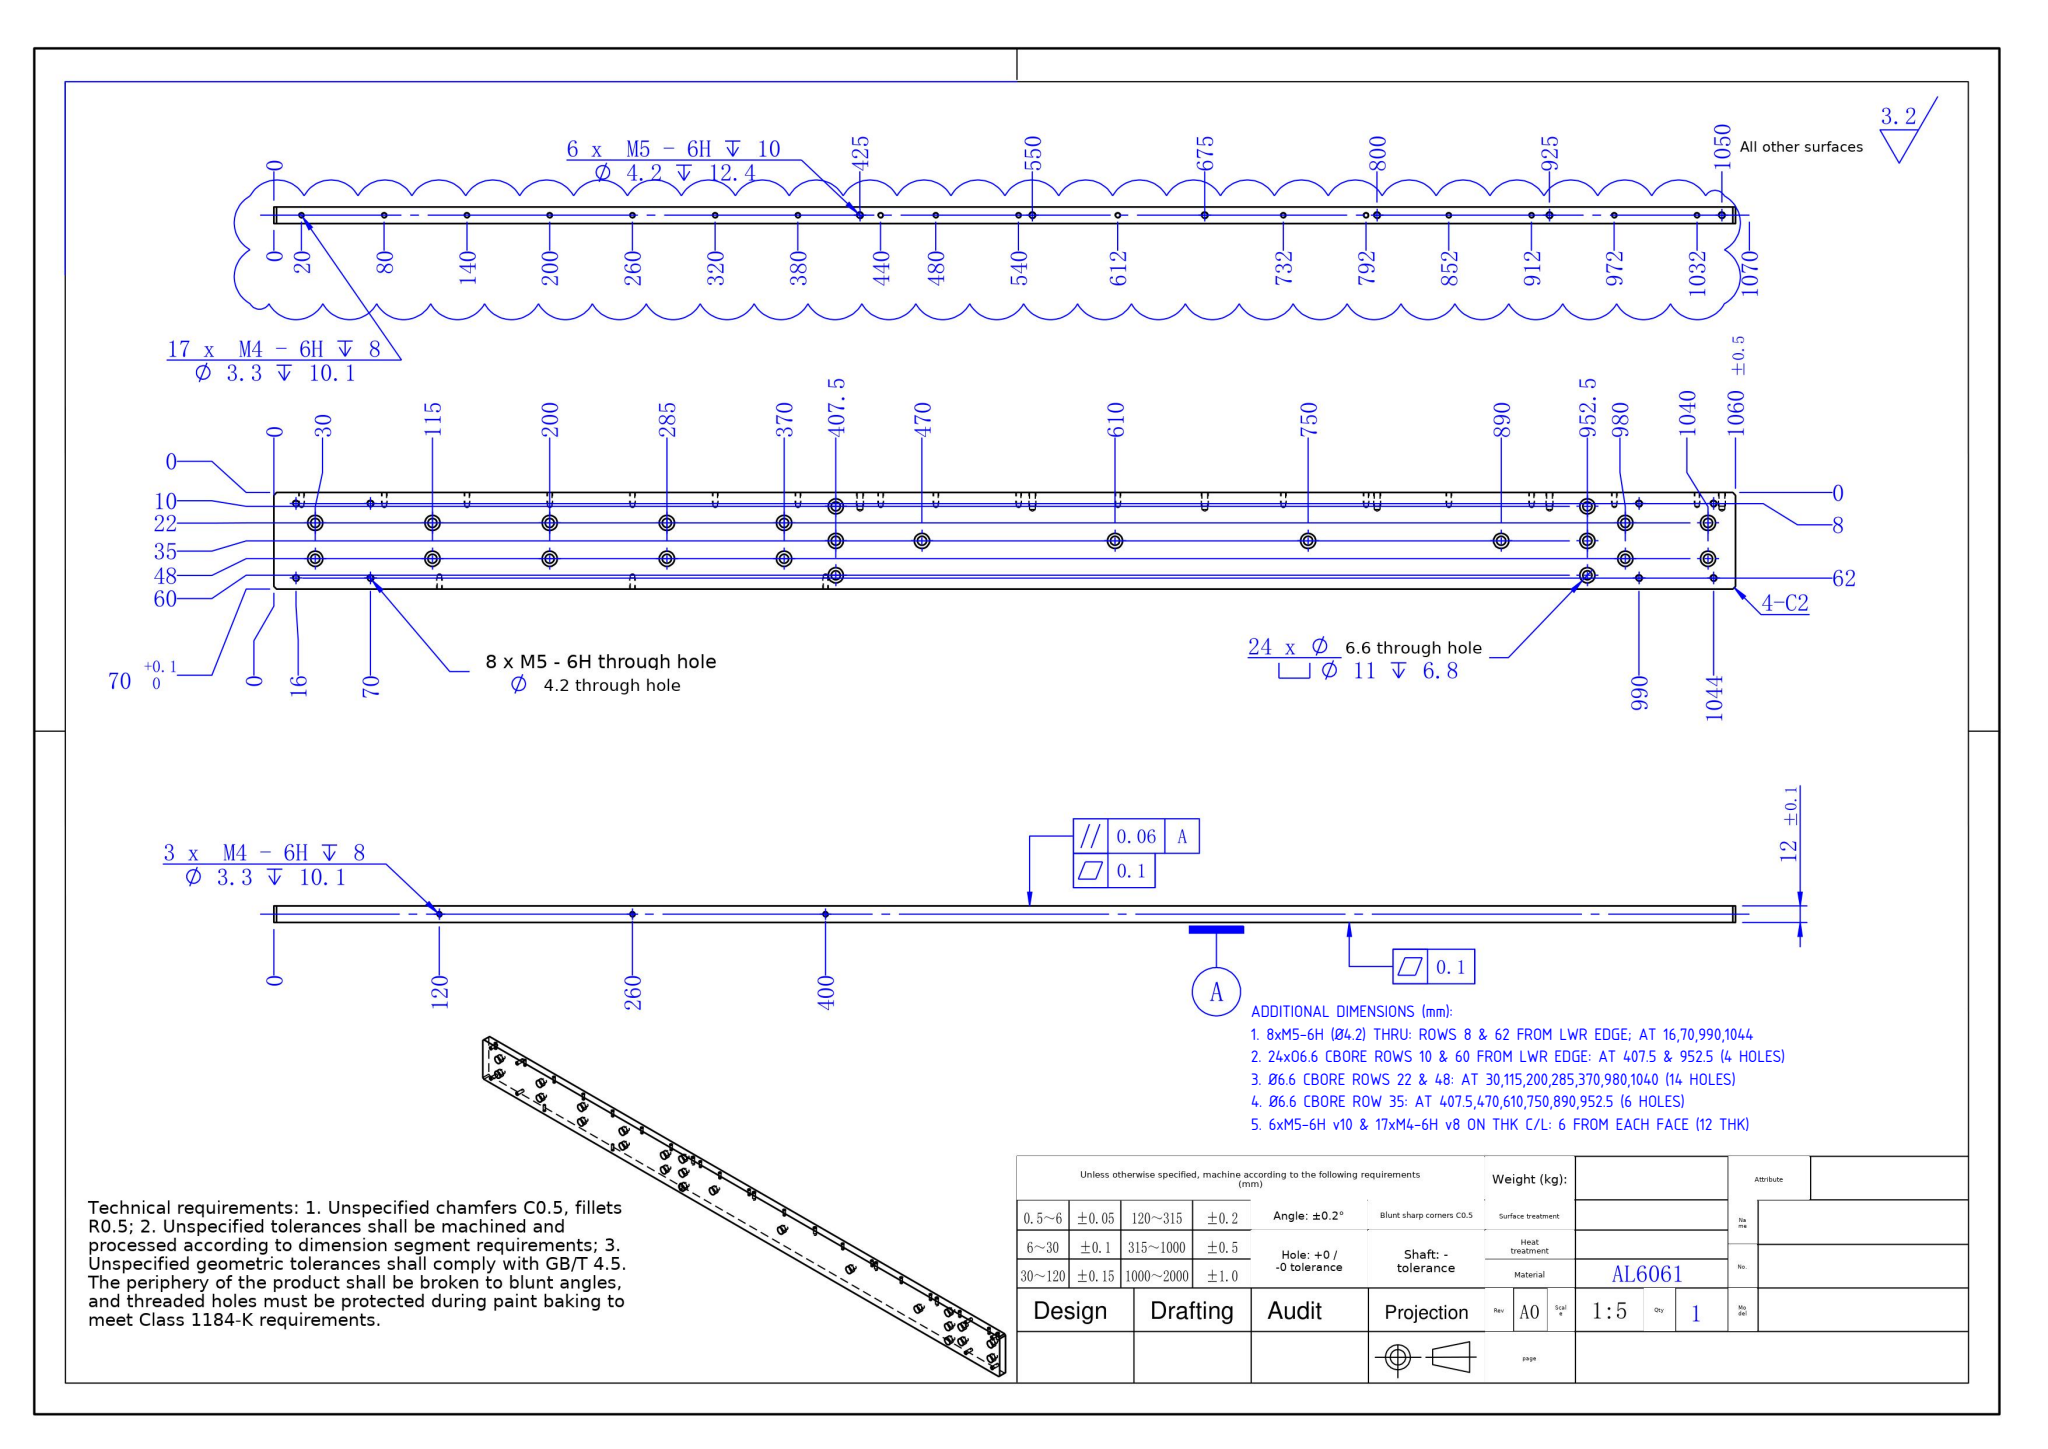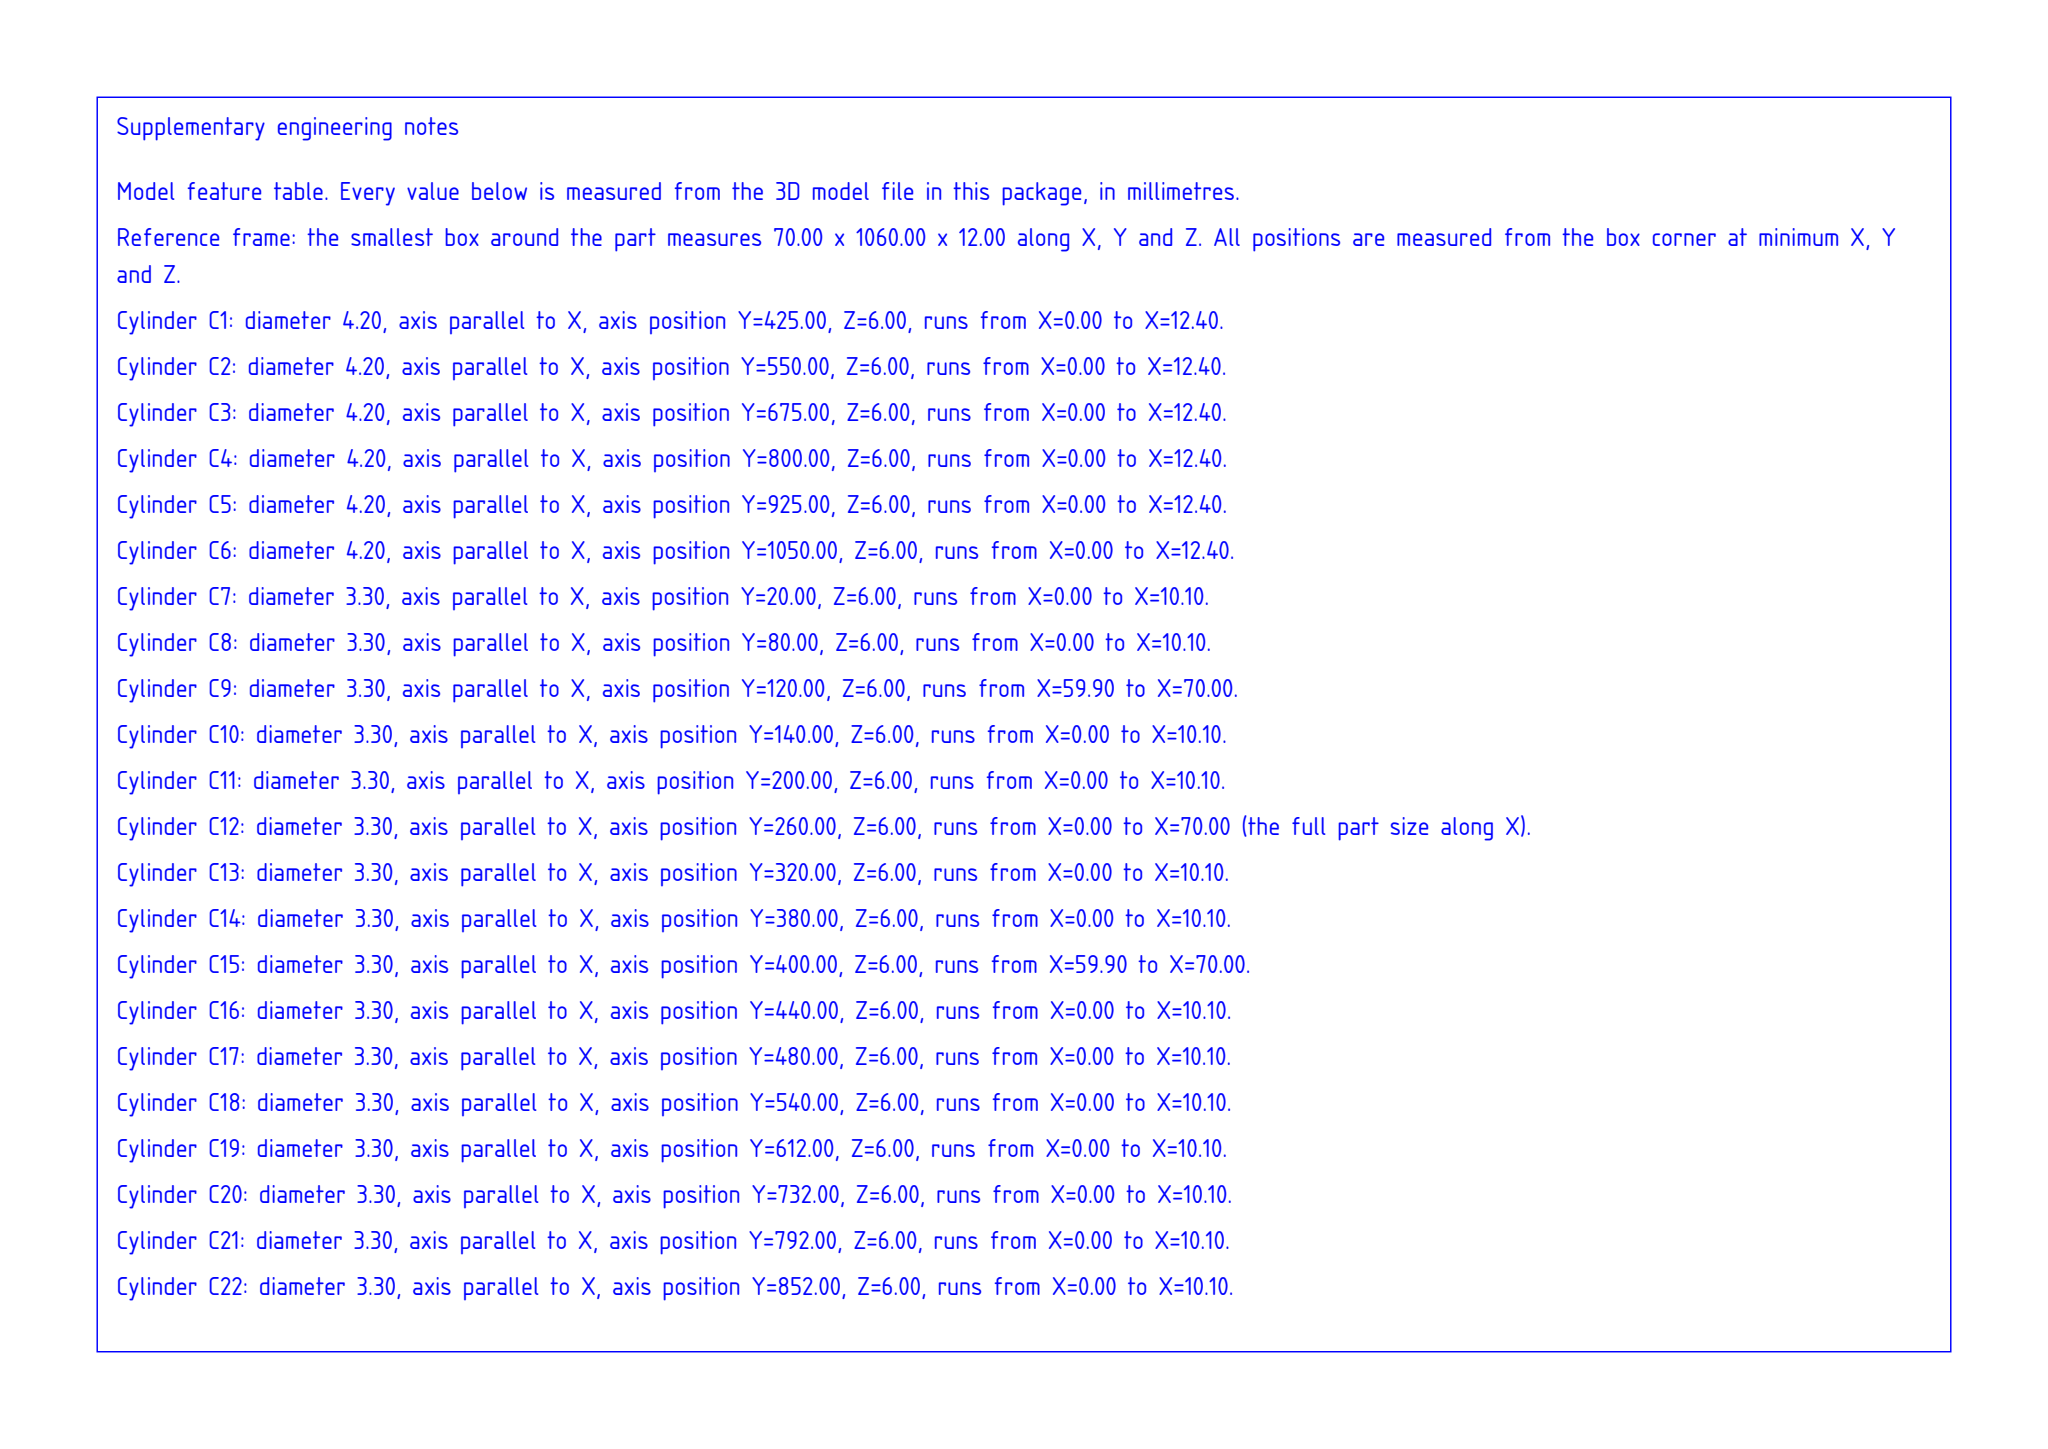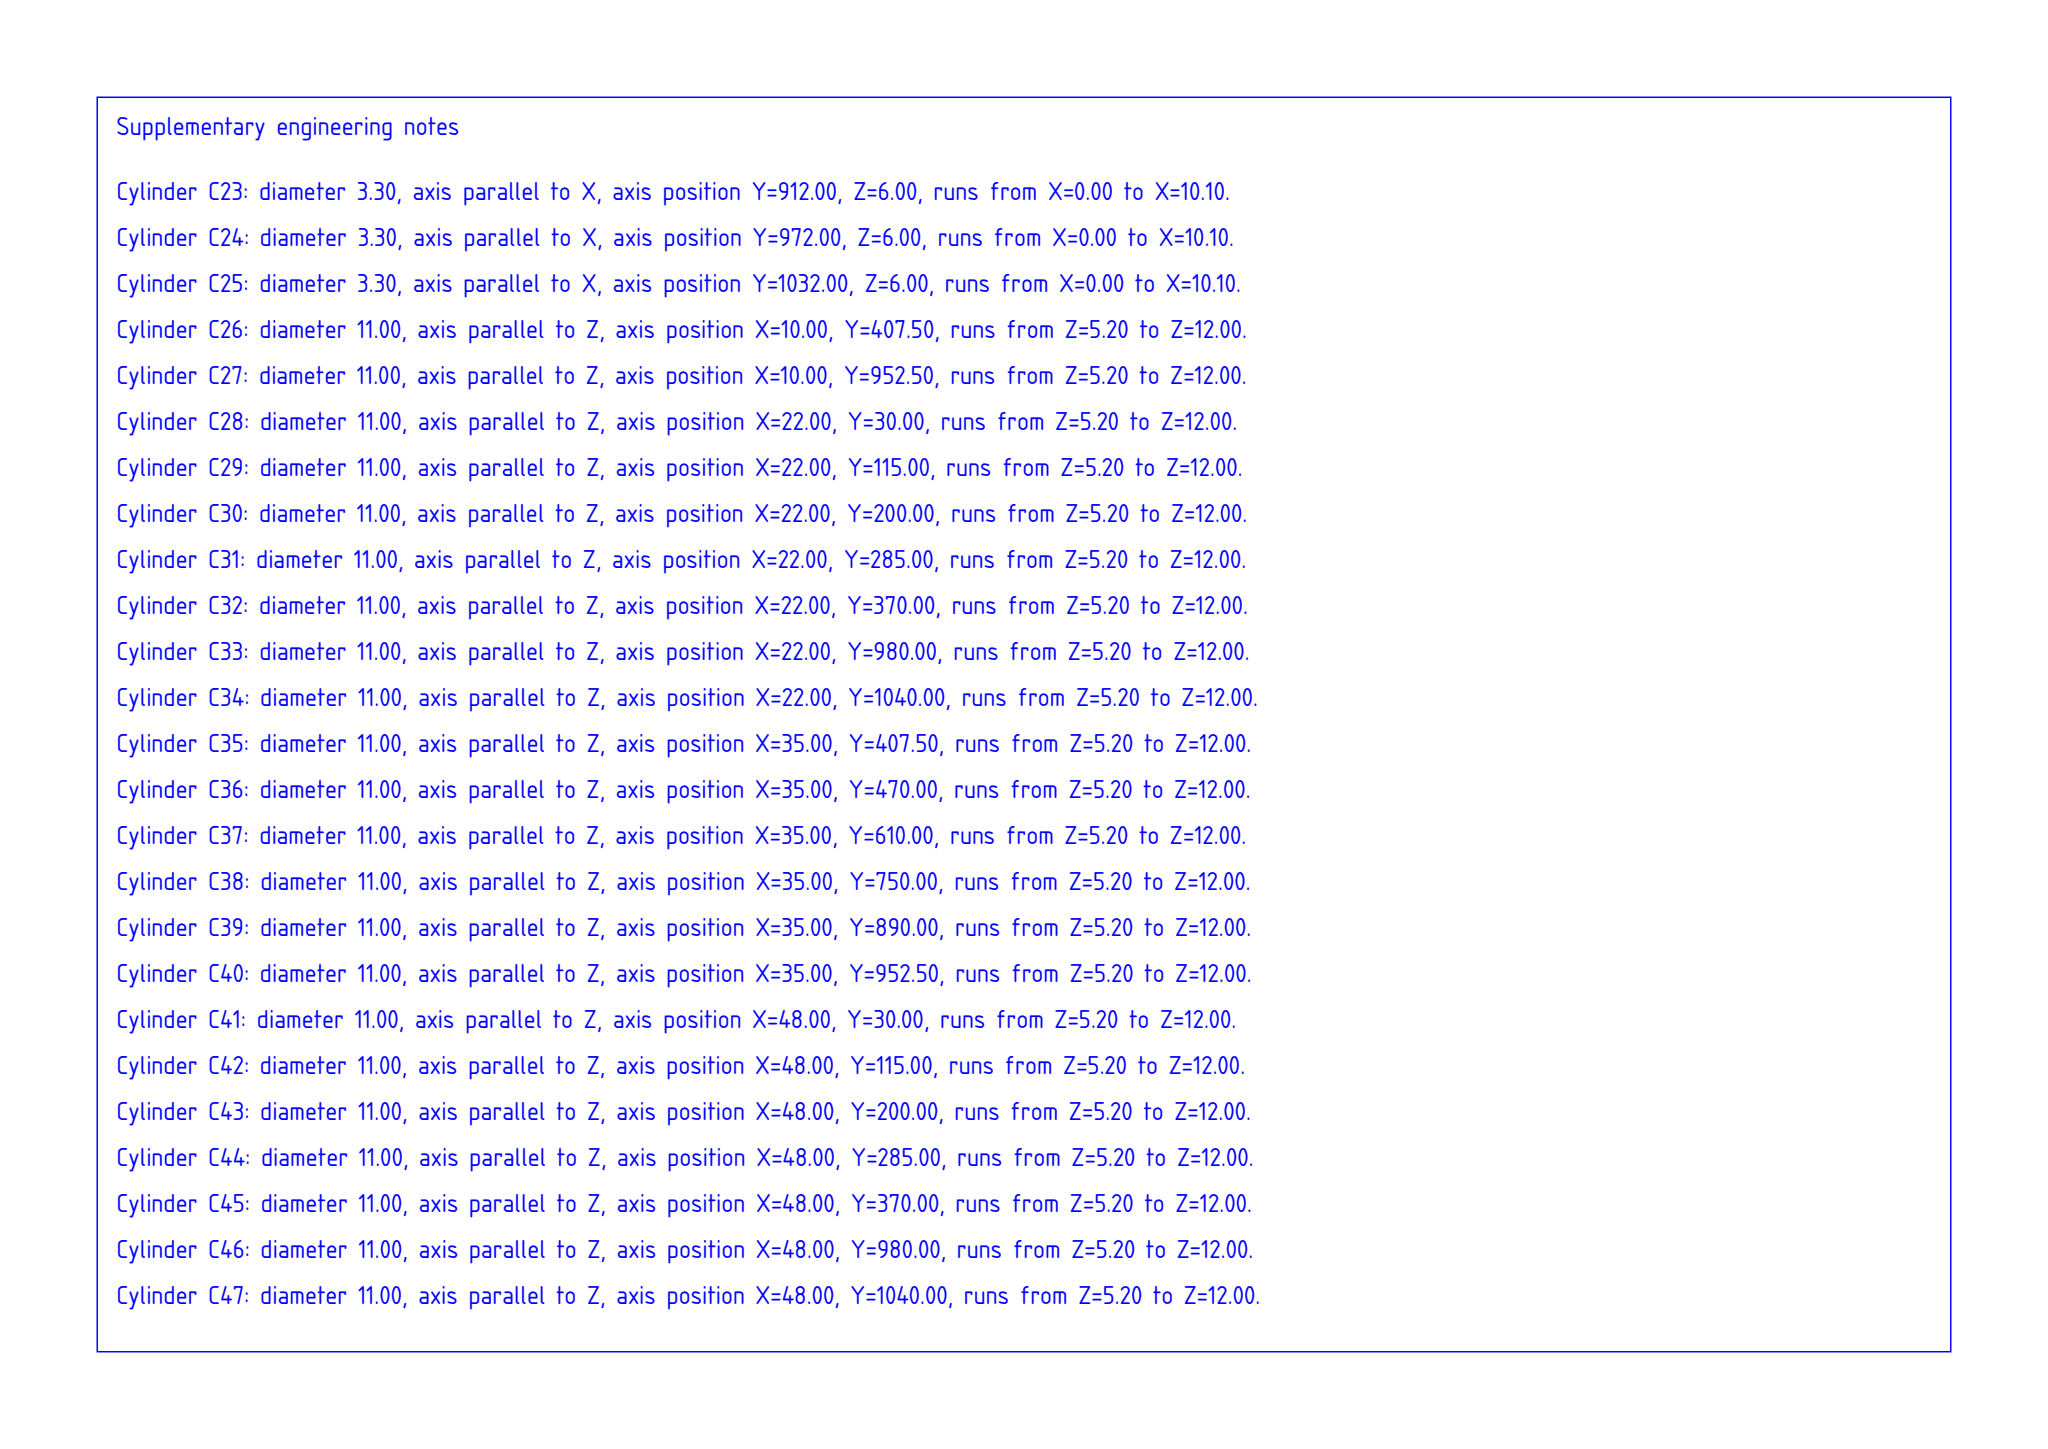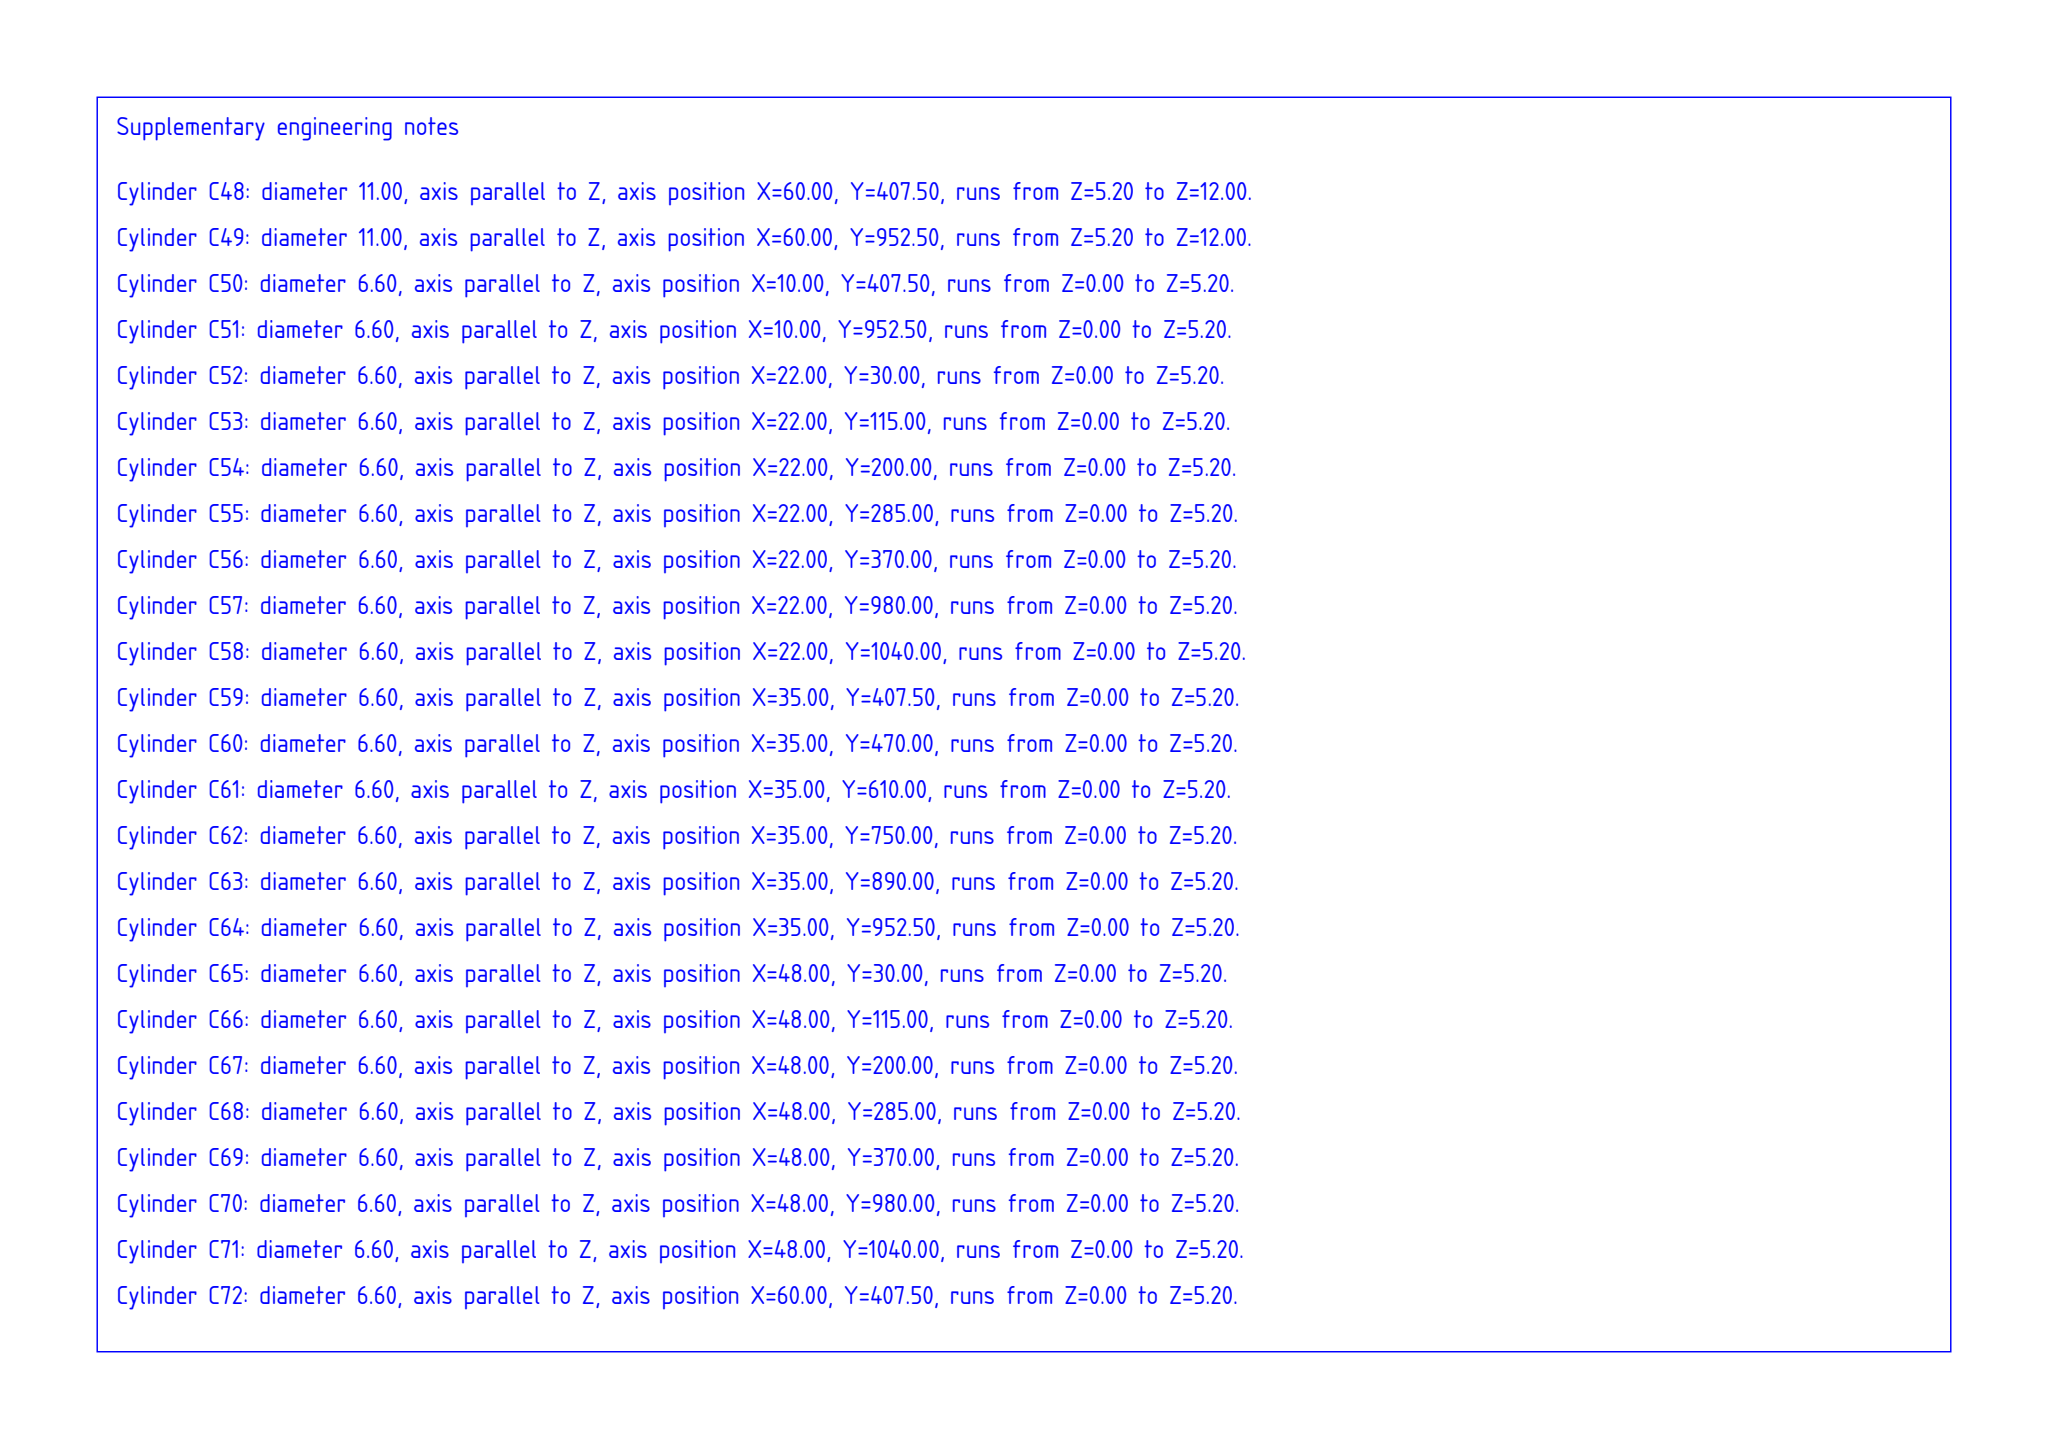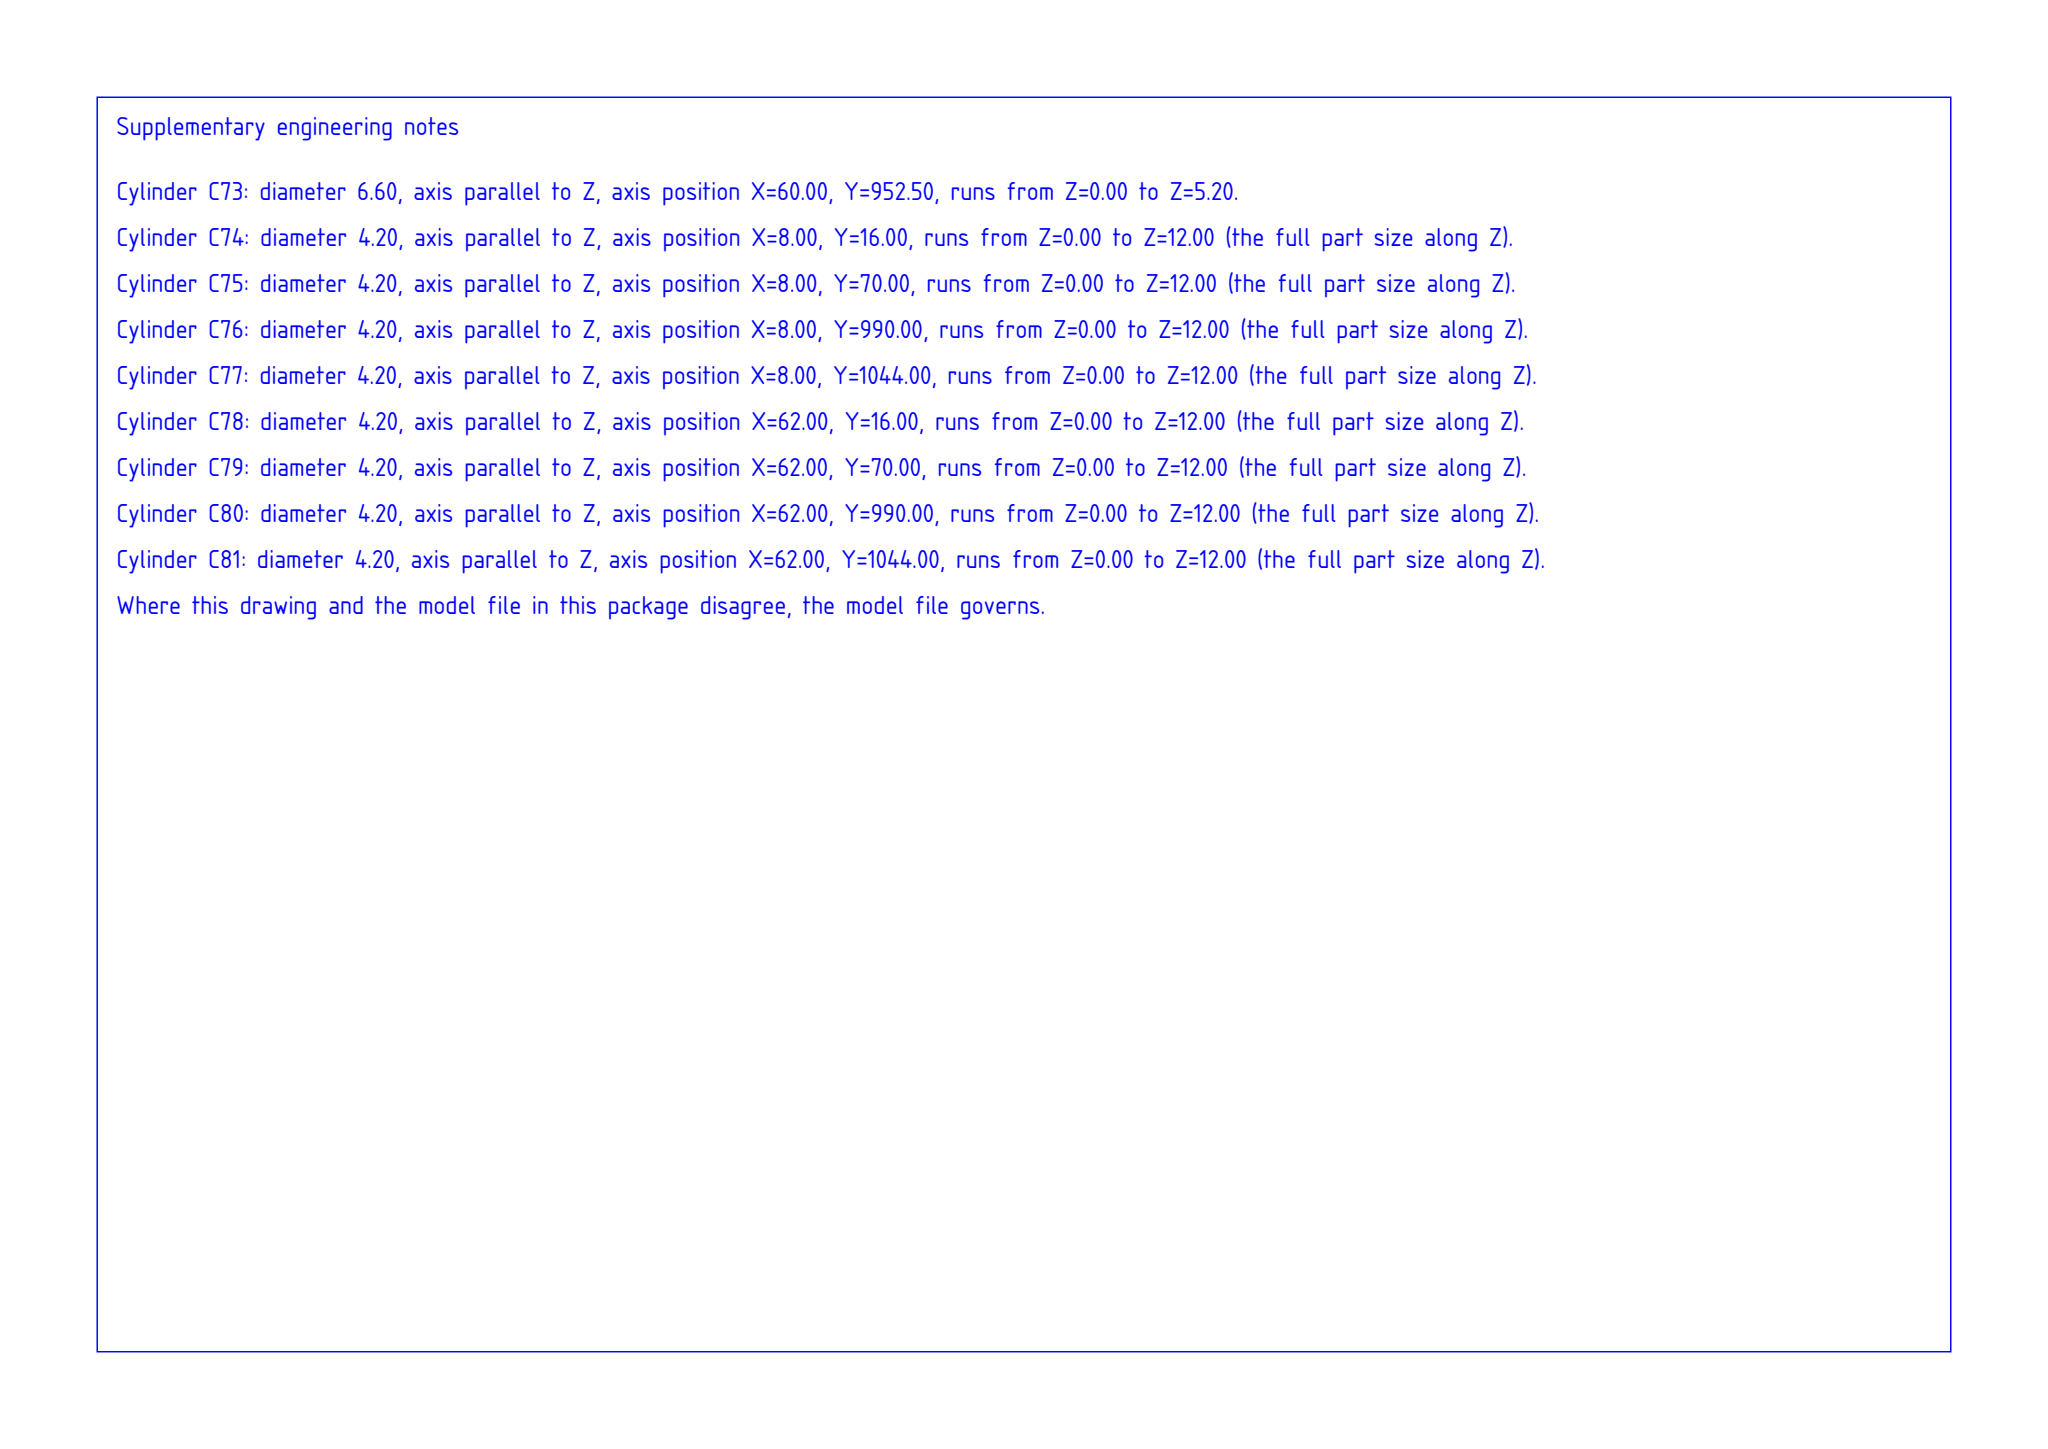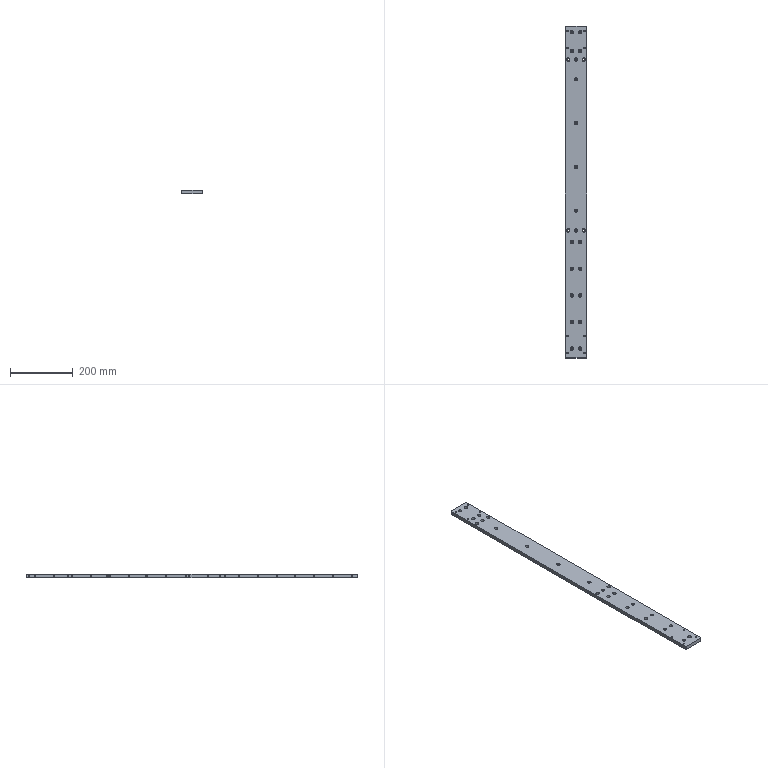Part | SolidWorks | mm | 1 solid | 250 faces | box 70 x 1060 x 12 mm | volume 866345 mm3 | cylinder 164 | cone 52 | plane 34 | commonest cylinder face diameters 11 x48 6.6 x48 3.3 x40 4.2 x28
build123d program:
from build123d import *

# Parameters (mm, degrees)
SKETCH1_W                                         = 70
SKETCH1_H                                         = 1060
BOSS_EXTRUDE1_DEPTH                               = 6
CHAMFER1_SIZE                                     = 2
M5_TAPPED_HOLE1_D                                 = 4.2
HOLE_SIZE_ACCORDING_TO_TYPE_0_OF_HEXA_D           = 6.6
HOLE_SIZE_ACCORDING_TO_TYPE_0_OF_HEXA_CBORE_D     = 11
HOLE_SIZE_ACCORDING_TO_TYPE_0_OF_HEXA_CBORE_DEPTH = 6.8
M4_TAPPED_HOLE1_D                                 = 3.3
M4_TAPPED_HOLE1_DEPTH                             = 10.1
M4_TAPPED_HOLE1_TIP                               = 0.9914
M5_TAPPED_HOLE2_D                                 = 4.2
M5_TAPPED_HOLE2_DEPTH                             = 12.4
M5_TAPPED_HOLE2_TIP                               = 1.262
M4_TAPPED_HOLE2_D                                 = 3.3
M4_TAPPED_HOLE2_DEPTH                             = 10.1
M4_TAPPED_HOLE2_TIP                               = 0.9914


with BuildPart() as part:
    # Sketch1 → Boss-Extrude1 (new, symmetric)
    with BuildSketch(Plane.XY):
        Rectangle(SKETCH1_W, SKETCH1_H)
    extrude(amount=BOSS_EXTRUDE1_DEPTH, both=True)

    # Chamfer1
    chamfer1_edges = [part.edges().sort_by_distance(p)[0] for p in [
        (35, -530, 0),
        (-35, -530, 0),
        (-35, 530, 0),
        (35, 530, 0),
    ]]
    chamfer(chamfer1_edges, length=CHAMFER1_SIZE)

    # M5 Tapped Hole1 (through all)
    with Locations(Plane.XY.offset(6)):
        with Locations((27, -514), (27, -460), (-27, -460), (-27, -514), (27, 514), (27, 460), (-27, 460), (-27, 514)):
            Hole(M5_TAPPED_HOLE1_D / 2)

    # Hole Size _ according to_ type 0 of Hexa (through all)
    with Locations(Plane.XY.offset(6)):
        with Locations((0, -60), (0, 80), (0, 360), (13, 510), (13, 450), (-13, -500), (-13, -415), (-13, -330), (-13, -245), (-13, -160), (13, -160), (13, -245), (13, -330), (13, -415), (13, -500), (-13, 450), (-13, 510), (-25, -122.5), (0, -122.5), (25, -122.5), (25, 422.5), (0, 422.5), (-25, 422.5), (0, 220)):
            CounterBoreHole(HOLE_SIZE_ACCORDING_TO_TYPE_0_OF_HEXA_D / 2, HOLE_SIZE_ACCORDING_TO_TYPE_0_OF_HEXA_CBORE_D / 2, HOLE_SIZE_ACCORDING_TO_TYPE_0_OF_HEXA_CBORE_DEPTH)

    # M4 Tapped Hole1
    with Locations(Plane(origin=(35, 0, 0), x_dir=(0, 0, -1), z_dir=(1, 0, 0))):
        with Locations((0, -410), (0, -270), (0, -130)):
            Hole(M4_TAPPED_HOLE1_D / 2, depth=M4_TAPPED_HOLE1_DEPTH)
            with Locations((0, 0, -(M4_TAPPED_HOLE1_DEPTH + M4_TAPPED_HOLE1_TIP / 2))):  # 118° drill point
                Cone(0, M4_TAPPED_HOLE1_D / 2, M4_TAPPED_HOLE1_TIP, mode=Mode.SUBTRACT)

    # M5 Tapped Hole2
    with Locations(Plane.ZY.offset(35)):
        with Locations((0, -105), (0, 20), (0, 145), (0, 270), (0, 395), (0, 520)):
            Hole(M5_TAPPED_HOLE2_D / 2, depth=M5_TAPPED_HOLE2_DEPTH)
            with Locations((0, 0, -(M5_TAPPED_HOLE2_DEPTH + M5_TAPPED_HOLE2_TIP / 2))):  # 118° drill point
                Cone(0, M5_TAPPED_HOLE2_D / 2, M5_TAPPED_HOLE2_TIP, mode=Mode.SUBTRACT)

    # M4 Tapped Hole2
    with Locations(Plane.ZY.offset(35)):
        with Locations((0.000004748, -510), (0.000004748, -450), (0.000004748, -390), (0.000004748, -330), (0.000004748, -270), (0.000004748, -210), (0.000004748, -150), (0.000004748, -90), (0.000004748, -50), (0.000004748, 10), (0.000004748, 82), (0.000004748, 202), (0.000004748, 262), (0.000004748, 322), (0.000004748, 382), (0.000004748, 442), (0.000004748, 502)):
            Hole(M4_TAPPED_HOLE2_D / 2, depth=M4_TAPPED_HOLE2_DEPTH)
            with Locations((0, 0, -(M4_TAPPED_HOLE2_DEPTH + M4_TAPPED_HOLE2_TIP / 2))):  # 118° drill point
                Cone(0, M4_TAPPED_HOLE2_D / 2, M4_TAPPED_HOLE2_TIP, mode=Mode.SUBTRACT)


solid = part.part